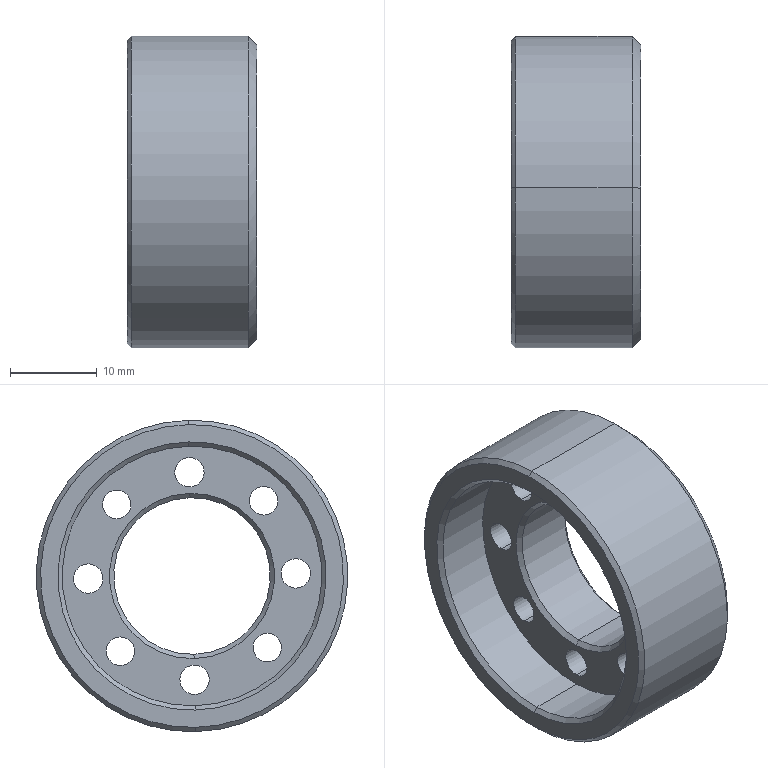Component | SolidWorks | JJDJR-3060-E-003-1 | 1 solid | 55 faces | volume 7393 mm3 | cylinder 30 | cone 18 | plane 7 | commonest cylinder face diameters 3.3 x8 5.5 x8 3.4 x8 30 x2 36 x2 18.1 x2 | material 45#